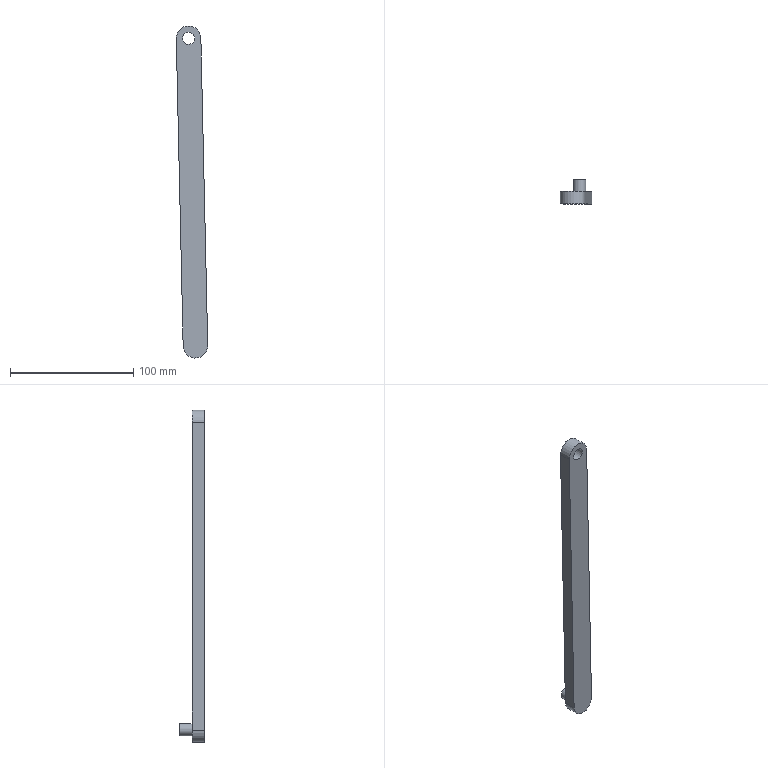Component | NX | 03 | 1 solid | 9 faces | box 25.59 x 20 x 269.94 mm | volume 53142 mm3 | plane 5 | cylinder 4 | commonest cylinder face diameters 20 x2 10 x2
STEP:
#1=CARTESIAN_POINT('',(0.,0.,0.));
#2=DIRECTION('',(0.,0.,1.));
#3=DIRECTION('',(1.,0.,0.));
#4=AXIS2_PLACEMENT_3D('',#1,#2,#3);
#5=CARTESIAN_POINT('',(208.953,15.,299.814));
#6=VERTEX_POINT('',#5);
#7=CARTESIAN_POINT('',(188.958,15.,299.367));
#8=VERTEX_POINT('',#7);
#9=CARTESIAN_POINT('',(198.956,15.,299.59));
#10=DIRECTION('',(0.,-1.,0.));
#11=DIRECTION('',(0.02235,0.,-0.9998));
#12=AXIS2_PLACEMENT_3D('',#9,#10,#11);
#13=CIRCLE('',#12,10.);
#14=CARTESIAN_POINT('',(198.956,5.,299.59));
#15=DIRECTION('',(0.,1.,0.));
#16=DIRECTION('',(0.9998,0.,0.02235));
#17=AXIS2_PLACEMENT_3D('',#14,#15,#16);
#18=CYLINDRICAL_SURFACE('',#17,10.);
#19=CARTESIAN_POINT('',(7.854,10.));
#20=DIRECTION('',(-1.,0.));
#21=VECTOR('',#20,1.);
#22=LINE('',#19,#21);
#23=(GEOMETRIC_REPRESENTATION_CONTEXT(2)PARAMETRIC_REPRESENTATION_CONTEXT()REPRESENTATION_CONTEXT('',''));
#24=DEFINITIONAL_REPRESENTATION('',(#22),#23);
#25=PCURVE('',#18,#24);
#26=CARTESIAN_POINT('',(198.956,15.,299.59));
#27=DIRECTION('',(0.,-1.,0.));
#28=DIRECTION('',(-0.9998,0.,-0.02235));
#29=AXIS2_PLACEMENT_3D('',#26,#27,#28);
#30=PLANE('',#29);
#31=CARTESIAN_POINT('',(0.,0.));
#32=DIRECTION('',(-0.,1.));
#33=AXIS2_PLACEMENT_2D('',#31,#32);
#34=CIRCLE('',#33,10.);
#35=(GEOMETRIC_REPRESENTATION_CONTEXT(2)PARAMETRIC_REPRESENTATION_CONTEXT()REPRESENTATION_CONTEXT('',''));
#36=DEFINITIONAL_REPRESENTATION('',(#34),#35);
#37=PCURVE('',#30,#36);
#38=SURFACE_CURVE('',#13,(#25,#37),.PCURVE_S1.);
#39=EDGE_CURVE('',#6,#8,#38,.T.);
#40=ORIENTED_EDGE('',*,*,#39,.T.);
#41=CARTESIAN_POINT('',(188.958,5.,299.367));
#42=VERTEX_POINT('',#41);
#43=CARTESIAN_POINT('',(188.958,5.,299.367));
#44=DIRECTION('',(0.,1.,0.));
#45=VECTOR('',#44,1.);
#46=LINE('',#43,#45);
#47=CARTESIAN_POINT('',(3.142,0.));
#48=DIRECTION('',(0.,1.));
#49=VECTOR('',#48,1.);
#50=LINE('',#47,#49);
#51=(GEOMETRIC_REPRESENTATION_CONTEXT(2)PARAMETRIC_REPRESENTATION_CONTEXT()REPRESENTATION_CONTEXT('',''));
#52=DEFINITIONAL_REPRESENTATION('',(#50),#51);
#53=PCURVE('',#18,#52);
#54=CARTESIAN_POINT('',(188.958,5.,299.367));
#55=DIRECTION('',(0.9998,0.,0.02235));
#56=DIRECTION('',(0.02235,0.,-0.9998));
#57=AXIS2_PLACEMENT_3D('',#54,#55,#56);
#58=PLANE('',#57);
#59=CARTESIAN_POINT('',(0.,0.));
#60=DIRECTION('',(0.,1.));
#61=VECTOR('',#60,1.);
#62=LINE('',#59,#61);
#63=(GEOMETRIC_REPRESENTATION_CONTEXT(2)PARAMETRIC_REPRESENTATION_CONTEXT()REPRESENTATION_CONTEXT('',''));
#64=DEFINITIONAL_REPRESENTATION('',(#62),#63);
#65=PCURVE('',#58,#64);
#66=SURFACE_CURVE('',#46,(#53,#65),.PCURVE_S1.);
#67=EDGE_CURVE('',#42,#8,#66,.T.);
#68=ORIENTED_EDGE('',*,*,#67,.F.);
#69=CARTESIAN_POINT('',(208.953,5.,299.814));
#70=VERTEX_POINT('',#69);
#71=CARTESIAN_POINT('',(198.956,5.,299.59));
#72=DIRECTION('',(0.,-1.,0.));
#73=DIRECTION('',(0.02235,0.,-0.9998));
#74=AXIS2_PLACEMENT_3D('',#71,#72,#73);
#75=CIRCLE('',#74,10.);
#76=CARTESIAN_POINT('',(7.854,0.));
#77=DIRECTION('',(-1.,0.));
#78=VECTOR('',#77,1.);
#79=LINE('',#76,#78);
#80=(GEOMETRIC_REPRESENTATION_CONTEXT(2)PARAMETRIC_REPRESENTATION_CONTEXT()REPRESENTATION_CONTEXT('',''));
#81=DEFINITIONAL_REPRESENTATION('',(#79),#80);
#82=PCURVE('',#18,#81);
#83=CARTESIAN_POINT('',(198.956,5.,299.59));
#84=DIRECTION('',(0.,-1.,0.));
#85=DIRECTION('',(-0.9998,0.,-0.02235));
#86=AXIS2_PLACEMENT_3D('',#83,#84,#85);
#87=PLANE('',#86);
#88=CARTESIAN_POINT('',(0.,0.));
#89=DIRECTION('',(-0.,1.));
#90=AXIS2_PLACEMENT_2D('',#88,#89);
#91=CIRCLE('',#90,10.);
#92=(GEOMETRIC_REPRESENTATION_CONTEXT(2)PARAMETRIC_REPRESENTATION_CONTEXT()REPRESENTATION_CONTEXT('',''));
#93=DEFINITIONAL_REPRESENTATION('',(#91),#92);
#94=PCURVE('',#87,#93);
#95=SURFACE_CURVE('',#75,(#82,#94),.PCURVE_S1.);
#96=EDGE_CURVE('',#70,#42,#95,.T.);
#97=ORIENTED_EDGE('',*,*,#96,.F.);
#98=CARTESIAN_POINT('',(208.953,5.,299.814));
#99=DIRECTION('',(0.,1.,0.));
#100=VECTOR('',#99,1.);
#101=LINE('',#98,#100);
#102=CARTESIAN_POINT('',(6.283,0.));
#103=DIRECTION('',(0.,1.));
#104=VECTOR('',#103,1.);
#105=LINE('',#102,#104);
#106=(GEOMETRIC_REPRESENTATION_CONTEXT(2)PARAMETRIC_REPRESENTATION_CONTEXT()REPRESENTATION_CONTEXT('',''));
#107=DEFINITIONAL_REPRESENTATION('',(#105),#106);
#108=PCURVE('',#18,#107);
#109=CARTESIAN_POINT('',(214.54,5.,49.876));
#110=DIRECTION('',(-0.9998,0.,-0.02235));
#111=DIRECTION('',(-0.02235,0.,0.9998));
#112=AXIS2_PLACEMENT_3D('',#109,#110,#111);
#113=PLANE('',#112);
#114=CARTESIAN_POINT('',(250.,0.));
#115=DIRECTION('',(0.,1.));
#116=VECTOR('',#115,1.);
#117=LINE('',#114,#116);
#118=(GEOMETRIC_REPRESENTATION_CONTEXT(2)PARAMETRIC_REPRESENTATION_CONTEXT()REPRESENTATION_CONTEXT('',''));
#119=DEFINITIONAL_REPRESENTATION('',(#117),#118);
#120=PCURVE('',#113,#119);
#121=SURFACE_CURVE('',#101,(#108,#120),.PCURVE_S1.);
#122=EDGE_CURVE('',#70,#6,#121,.T.);
#123=ORIENTED_EDGE('',*,*,#122,.T.);
#124=EDGE_LOOP('',(#40,#68,#97,#123));
#125=FACE_BOUND('',#124,.T.);
#126=ADVANCED_FACE('',(#125),#18,.T.);
#127=CARTESIAN_POINT('',(194.545,15.,49.429));
#128=VERTEX_POINT('',#127);
#129=CARTESIAN_POINT('',(188.958,15.,299.367));
#130=DIRECTION('',(0.02235,0.,-0.9998));
#131=VECTOR('',#130,1.);
#132=LINE('',#129,#131);
#133=CARTESIAN_POINT('',(0.,10.));
#134=DIRECTION('',(1.,0.));
#135=VECTOR('',#134,1.);
#136=LINE('',#133,#135);
#137=(GEOMETRIC_REPRESENTATION_CONTEXT(2)PARAMETRIC_REPRESENTATION_CONTEXT()REPRESENTATION_CONTEXT('',''));
#138=DEFINITIONAL_REPRESENTATION('',(#136),#137);
#139=PCURVE('',#58,#138);
#140=CARTESIAN_POINT('',(10.,-0.));
#141=DIRECTION('',(0.,1.));
#142=VECTOR('',#141,1.);
#143=LINE('',#140,#142);
#144=(GEOMETRIC_REPRESENTATION_CONTEXT(2)PARAMETRIC_REPRESENTATION_CONTEXT()REPRESENTATION_CONTEXT('',''));
#145=DEFINITIONAL_REPRESENTATION('',(#143),#144);
#146=PCURVE('',#30,#145);
#147=SURFACE_CURVE('',#132,(#139,#146),.PCURVE_S1.);
#148=EDGE_CURVE('',#8,#128,#147,.T.);
#149=ORIENTED_EDGE('',*,*,#148,.T.);
#150=CARTESIAN_POINT('',(194.545,5.,49.429));
#151=VERTEX_POINT('',#150);
#152=CARTESIAN_POINT('',(194.545,5.,49.429));
#153=DIRECTION('',(0.,1.,0.));
#154=VECTOR('',#153,1.);
#155=LINE('',#152,#154);
#156=CARTESIAN_POINT('',(250.,0.));
#157=DIRECTION('',(0.,1.));
#158=VECTOR('',#157,1.);
#159=LINE('',#156,#158);
#160=(GEOMETRIC_REPRESENTATION_CONTEXT(2)PARAMETRIC_REPRESENTATION_CONTEXT()REPRESENTATION_CONTEXT('',''));
#161=DEFINITIONAL_REPRESENTATION('',(#159),#160);
#162=PCURVE('',#58,#161);
#163=CARTESIAN_POINT('',(204.543,5.,49.653));
#164=DIRECTION('',(0.,1.,0.));
#165=DIRECTION('',(0.9998,0.,0.02235));
#166=AXIS2_PLACEMENT_3D('',#163,#164,#165);
#167=CYLINDRICAL_SURFACE('',#166,10.);
#168=CARTESIAN_POINT('',(3.142,0.));
#169=DIRECTION('',(0.,1.));
#170=VECTOR('',#169,1.);
#171=LINE('',#168,#170);
#172=(GEOMETRIC_REPRESENTATION_CONTEXT(2)PARAMETRIC_REPRESENTATION_CONTEXT()REPRESENTATION_CONTEXT('',''));
#173=DEFINITIONAL_REPRESENTATION('',(#171),#172);
#174=PCURVE('',#167,#173);
#175=SURFACE_CURVE('',#155,(#162,#174),.PCURVE_S1.);
#176=EDGE_CURVE('',#151,#128,#175,.T.);
#177=ORIENTED_EDGE('',*,*,#176,.F.);
#178=CARTESIAN_POINT('',(188.958,5.,299.367));
#179=DIRECTION('',(0.02235,0.,-0.9998));
#180=VECTOR('',#179,1.);
#181=LINE('',#178,#180);
#182=CARTESIAN_POINT('',(0.,0.));
#183=DIRECTION('',(1.,0.));
#184=VECTOR('',#183,1.);
#185=LINE('',#182,#184);
#186=(GEOMETRIC_REPRESENTATION_CONTEXT(2)PARAMETRIC_REPRESENTATION_CONTEXT()REPRESENTATION_CONTEXT('',''));
#187=DEFINITIONAL_REPRESENTATION('',(#185),#186);
#188=PCURVE('',#58,#187);
#189=CARTESIAN_POINT('',(10.,-0.));
#190=DIRECTION('',(0.,1.));
#191=VECTOR('',#190,1.);
#192=LINE('',#189,#191);
#193=(GEOMETRIC_REPRESENTATION_CONTEXT(2)PARAMETRIC_REPRESENTATION_CONTEXT()REPRESENTATION_CONTEXT('',''));
#194=DEFINITIONAL_REPRESENTATION('',(#192),#193);
#195=PCURVE('',#87,#194);
#196=SURFACE_CURVE('',#181,(#188,#195),.PCURVE_S1.);
#197=EDGE_CURVE('',#42,#151,#196,.T.);
#198=ORIENTED_EDGE('',*,*,#197,.F.);
#199=ORIENTED_EDGE('',*,*,#67,.T.);
#200=EDGE_LOOP('',(#149,#177,#198,#199));
#201=FACE_BOUND('',#200,.T.);
#202=ADVANCED_FACE('',(#201),#58,.F.);
#203=CARTESIAN_POINT('',(214.54,15.,49.876));
#204=VERTEX_POINT('',#203);
#205=CARTESIAN_POINT('',(204.543,15.,49.653));
#206=DIRECTION('',(0.,-1.,0.));
#207=DIRECTION('',(0.02235,0.,-0.9998));
#208=AXIS2_PLACEMENT_3D('',#205,#206,#207);
#209=CIRCLE('',#208,10.);
#210=CARTESIAN_POINT('',(7.854,10.));
#211=DIRECTION('',(-1.,0.));
#212=VECTOR('',#211,1.);
#213=LINE('',#210,#212);
#214=(GEOMETRIC_REPRESENTATION_CONTEXT(2)PARAMETRIC_REPRESENTATION_CONTEXT()REPRESENTATION_CONTEXT('',''));
#215=DEFINITIONAL_REPRESENTATION('',(#213),#214);
#216=PCURVE('',#167,#215);
#217=CARTESIAN_POINT('',(0.,250.));
#218=DIRECTION('',(-0.,1.));
#219=AXIS2_PLACEMENT_2D('',#217,#218);
#220=CIRCLE('',#219,10.);
#221=(GEOMETRIC_REPRESENTATION_CONTEXT(2)PARAMETRIC_REPRESENTATION_CONTEXT()REPRESENTATION_CONTEXT('',''));
#222=DEFINITIONAL_REPRESENTATION('',(#220),#221);
#223=PCURVE('',#30,#222);
#224=SURFACE_CURVE('',#209,(#216,#223),.PCURVE_S1.);
#225=EDGE_CURVE('',#128,#204,#224,.T.);
#226=ORIENTED_EDGE('',*,*,#225,.T.);
#227=CARTESIAN_POINT('',(214.54,5.,49.876));
#228=VERTEX_POINT('',#227);
#229=CARTESIAN_POINT('',(214.54,5.,49.876));
#230=DIRECTION('',(0.,1.,0.));
#231=VECTOR('',#230,1.);
#232=LINE('',#229,#231);
#233=CARTESIAN_POINT('',(0.,0.));
#234=DIRECTION('',(0.,1.));
#235=VECTOR('',#234,1.);
#236=LINE('',#233,#235);
#237=(GEOMETRIC_REPRESENTATION_CONTEXT(2)PARAMETRIC_REPRESENTATION_CONTEXT()REPRESENTATION_CONTEXT('',''));
#238=DEFINITIONAL_REPRESENTATION('',(#236),#237);
#239=PCURVE('',#167,#238);
#240=CARTESIAN_POINT('',(0.,0.));
#241=DIRECTION('',(0.,1.));
#242=VECTOR('',#241,1.);
#243=LINE('',#240,#242);
#244=(GEOMETRIC_REPRESENTATION_CONTEXT(2)PARAMETRIC_REPRESENTATION_CONTEXT()REPRESENTATION_CONTEXT('',''));
#245=DEFINITIONAL_REPRESENTATION('',(#243),#244);
#246=PCURVE('',#113,#245);
#247=SURFACE_CURVE('',#232,(#239,#246),.PCURVE_S1.);
#248=EDGE_CURVE('',#228,#204,#247,.T.);
#249=ORIENTED_EDGE('',*,*,#248,.F.);
#250=CARTESIAN_POINT('',(204.543,5.,49.653));
#251=DIRECTION('',(0.,-1.,0.));
#252=DIRECTION('',(0.02235,0.,-0.9998));
#253=AXIS2_PLACEMENT_3D('',#250,#251,#252);
#254=CIRCLE('',#253,10.);
#255=CARTESIAN_POINT('',(7.854,0.));
#256=DIRECTION('',(-1.,0.));
#257=VECTOR('',#256,1.);
#258=LINE('',#255,#257);
#259=(GEOMETRIC_REPRESENTATION_CONTEXT(2)PARAMETRIC_REPRESENTATION_CONTEXT()REPRESENTATION_CONTEXT('',''));
#260=DEFINITIONAL_REPRESENTATION('',(#258),#259);
#261=PCURVE('',#167,#260);
#262=CARTESIAN_POINT('',(0.,250.));
#263=DIRECTION('',(-0.,1.));
#264=AXIS2_PLACEMENT_2D('',#262,#263);
#265=CIRCLE('',#264,10.);
#266=(GEOMETRIC_REPRESENTATION_CONTEXT(2)PARAMETRIC_REPRESENTATION_CONTEXT()REPRESENTATION_CONTEXT('',''));
#267=DEFINITIONAL_REPRESENTATION('',(#265),#266);
#268=PCURVE('',#87,#267);
#269=SURFACE_CURVE('',#254,(#261,#268),.PCURVE_S1.);
#270=EDGE_CURVE('',#151,#228,#269,.T.);
#271=ORIENTED_EDGE('',*,*,#270,.F.);
#272=ORIENTED_EDGE('',*,*,#176,.T.);
#273=EDGE_LOOP('',(#226,#249,#271,#272));
#274=FACE_BOUND('',#273,.T.);
#275=ADVANCED_FACE('',(#274),#167,.T.);
#276=CARTESIAN_POINT('',(214.54,15.,49.876));
#277=DIRECTION('',(-0.02235,0.,0.9998));
#278=VECTOR('',#277,1.);
#279=LINE('',#276,#278);
#280=CARTESIAN_POINT('',(0.,10.));
#281=DIRECTION('',(1.,0.));
#282=VECTOR('',#281,1.);
#283=LINE('',#280,#282);
#284=(GEOMETRIC_REPRESENTATION_CONTEXT(2)PARAMETRIC_REPRESENTATION_CONTEXT()REPRESENTATION_CONTEXT('',''));
#285=DEFINITIONAL_REPRESENTATION('',(#283),#284);
#286=PCURVE('',#113,#285);
#287=CARTESIAN_POINT('',(-10.,250.));
#288=DIRECTION('',(0.,-1.));
#289=VECTOR('',#288,1.);
#290=LINE('',#287,#289);
#291=(GEOMETRIC_REPRESENTATION_CONTEXT(2)PARAMETRIC_REPRESENTATION_CONTEXT()REPRESENTATION_CONTEXT('',''));
#292=DEFINITIONAL_REPRESENTATION('',(#290),#291);
#293=PCURVE('',#30,#292);
#294=SURFACE_CURVE('',#279,(#286,#293),.PCURVE_S1.);
#295=EDGE_CURVE('',#204,#6,#294,.T.);
#296=ORIENTED_EDGE('',*,*,#295,.T.);
#297=ORIENTED_EDGE('',*,*,#122,.F.);
#298=CARTESIAN_POINT('',(214.54,5.,49.876));
#299=DIRECTION('',(-0.02235,0.,0.9998));
#300=VECTOR('',#299,1.);
#301=LINE('',#298,#300);
#302=CARTESIAN_POINT('',(0.,0.));
#303=DIRECTION('',(1.,0.));
#304=VECTOR('',#303,1.);
#305=LINE('',#302,#304);
#306=(GEOMETRIC_REPRESENTATION_CONTEXT(2)PARAMETRIC_REPRESENTATION_CONTEXT()REPRESENTATION_CONTEXT('',''));
#307=DEFINITIONAL_REPRESENTATION('',(#305),#306);
#308=PCURVE('',#113,#307);
#309=CARTESIAN_POINT('',(-10.,250.));
#310=DIRECTION('',(0.,-1.));
#311=VECTOR('',#310,1.);
#312=LINE('',#309,#311);
#313=(GEOMETRIC_REPRESENTATION_CONTEXT(2)PARAMETRIC_REPRESENTATION_CONTEXT()REPRESENTATION_CONTEXT('',''));
#314=DEFINITIONAL_REPRESENTATION('',(#312),#313);
#315=PCURVE('',#87,#314);
#316=SURFACE_CURVE('',#301,(#308,#315),.PCURVE_S1.);
#317=EDGE_CURVE('',#228,#70,#316,.T.);
#318=ORIENTED_EDGE('',*,*,#317,.F.);
#319=ORIENTED_EDGE('',*,*,#248,.T.);
#320=EDGE_LOOP('',(#296,#297,#318,#319));
#321=FACE_BOUND('',#320,.T.);
#322=ADVANCED_FACE('',(#321),#113,.F.);
#323=CARTESIAN_POINT('',(193.957,5.,299.479));
#324=VERTEX_POINT('',#323);
#325=CARTESIAN_POINT('',(198.956,5.,299.59));
#326=DIRECTION('',(0.,-1.,0.));
#327=DIRECTION('',(-0.9998,0.,-0.02235));
#328=AXIS2_PLACEMENT_3D('',#325,#326,#327);
#329=CIRCLE('',#328,5.);
#330=CARTESIAN_POINT('',(0.,0.));
#331=DIRECTION('',(1.,0.));
#332=AXIS2_PLACEMENT_2D('',#330,#331);
#333=CIRCLE('',#332,5.);
#334=(GEOMETRIC_REPRESENTATION_CONTEXT(2)PARAMETRIC_REPRESENTATION_CONTEXT()REPRESENTATION_CONTEXT('',''));
#335=DEFINITIONAL_REPRESENTATION('',(#333),#334);
#336=PCURVE('',#87,#335);
#337=CARTESIAN_POINT('',(198.956,4.,299.59));
#338=DIRECTION('',(0.,1.,0.));
#339=DIRECTION('',(0.02235,0.,-0.9998));
#340=AXIS2_PLACEMENT_3D('',#337,#338,#339);
#341=CYLINDRICAL_SURFACE('',#340,5.);
#342=CARTESIAN_POINT('',(7.854,1.));
#343=DIRECTION('',(-1.,0.));
#344=VECTOR('',#343,1.);
#345=LINE('',#342,#344);
#346=(GEOMETRIC_REPRESENTATION_CONTEXT(2)PARAMETRIC_REPRESENTATION_CONTEXT()REPRESENTATION_CONTEXT('',''));
#347=DEFINITIONAL_REPRESENTATION('',(#345),#346);
#348=PCURVE('',#341,#347);
#349=SURFACE_CURVE('',#329,(#336,#348),.PCURVE_S1.);
#350=EDGE_CURVE('',#324,#324,#349,.T.);
#351=ORIENTED_EDGE('',*,*,#350,.F.);
#352=EDGE_LOOP('',(#351));
#353=FACE_BOUND('',#352,.T.);
#354=ORIENTED_EDGE('',*,*,#96,.T.);
#355=ORIENTED_EDGE('',*,*,#197,.T.);
#356=ORIENTED_EDGE('',*,*,#270,.T.);
#357=ORIENTED_EDGE('',*,*,#317,.T.);
#358=EDGE_LOOP('',(#354,#355,#356,#357));
#359=FACE_BOUND('',#358,.T.);
#360=ADVANCED_FACE('',(#353,#359),#87,.T.);
#361=CARTESIAN_POINT('',(204.431,15.,54.652));
#362=VERTEX_POINT('',#361);
#363=CARTESIAN_POINT('',(204.543,15.,49.653));
#364=DIRECTION('',(0.,-1.,0.));
#365=DIRECTION('',(-0.02235,0.,0.9998));
#366=AXIS2_PLACEMENT_3D('',#363,#364,#365);
#367=CIRCLE('',#366,5.);
#368=CARTESIAN_POINT('',(0.,250.));
#369=DIRECTION('',(0.,-1.));
#370=AXIS2_PLACEMENT_2D('',#368,#369);
#371=CIRCLE('',#370,5.);
#372=(GEOMETRIC_REPRESENTATION_CONTEXT(2)PARAMETRIC_REPRESENTATION_CONTEXT()REPRESENTATION_CONTEXT('',''));
#373=DEFINITIONAL_REPRESENTATION('',(#371),#372);
#374=PCURVE('',#30,#373);
#375=CARTESIAN_POINT('',(204.543,25.,49.653));
#376=DIRECTION('',(0.,-1.,0.));
#377=DIRECTION('',(-0.9998,0.,-0.02235));
#378=AXIS2_PLACEMENT_3D('',#375,#376,#377);
#379=CYLINDRICAL_SURFACE('',#378,5.);
#380=CARTESIAN_POINT('',(4.712,10.));
#381=DIRECTION('',(1.,0.));
#382=VECTOR('',#381,1.);
#383=LINE('',#380,#382);
#384=(GEOMETRIC_REPRESENTATION_CONTEXT(2)PARAMETRIC_REPRESENTATION_CONTEXT()REPRESENTATION_CONTEXT('',''));
#385=DEFINITIONAL_REPRESENTATION('',(#383),#384);
#386=PCURVE('',#379,#385);
#387=SURFACE_CURVE('',#367,(#374,#386),.PCURVE_S1.);
#388=EDGE_CURVE('',#362,#362,#387,.T.);
#389=ORIENTED_EDGE('',*,*,#388,.T.);
#390=EDGE_LOOP('',(#389));
#391=FACE_BOUND('',#390,.T.);
#392=CARTESIAN_POINT('',(193.957,15.,299.479));
#393=VERTEX_POINT('',#392);
#394=CARTESIAN_POINT('',(198.956,15.,299.59));
#395=DIRECTION('',(0.,-1.,0.));
#396=DIRECTION('',(-0.9998,0.,-0.02235));
#397=AXIS2_PLACEMENT_3D('',#394,#395,#396);
#398=CIRCLE('',#397,5.);
#399=CARTESIAN_POINT('',(0.,0.));
#400=DIRECTION('',(1.,0.));
#401=AXIS2_PLACEMENT_2D('',#399,#400);
#402=CIRCLE('',#401,5.);
#403=(GEOMETRIC_REPRESENTATION_CONTEXT(2)PARAMETRIC_REPRESENTATION_CONTEXT()REPRESENTATION_CONTEXT('',''));
#404=DEFINITIONAL_REPRESENTATION('',(#402),#403);
#405=PCURVE('',#30,#404);
#406=CARTESIAN_POINT('',(7.854,11.));
#407=DIRECTION('',(-1.,0.));
#408=VECTOR('',#407,1.);
#409=LINE('',#406,#408);
#410=(GEOMETRIC_REPRESENTATION_CONTEXT(2)PARAMETRIC_REPRESENTATION_CONTEXT()REPRESENTATION_CONTEXT('',''));
#411=DEFINITIONAL_REPRESENTATION('',(#409),#410);
#412=PCURVE('',#341,#411);
#413=SURFACE_CURVE('',#398,(#405,#412),.PCURVE_S1.);
#414=EDGE_CURVE('',#393,#393,#413,.T.);
#415=ORIENTED_EDGE('',*,*,#414,.T.);
#416=EDGE_LOOP('',(#415));
#417=FACE_BOUND('',#416,.T.);
#418=ORIENTED_EDGE('',*,*,#39,.F.);
#419=ORIENTED_EDGE('',*,*,#295,.F.);
#420=ORIENTED_EDGE('',*,*,#225,.F.);
#421=ORIENTED_EDGE('',*,*,#148,.F.);
#422=EDGE_LOOP('',(#418,#419,#420,#421));
#423=FACE_BOUND('',#422,.T.);
#424=ADVANCED_FACE('',(#391,#417,#423),#30,.F.);
#425=CARTESIAN_POINT('',(204.431,25.,54.652));
#426=VERTEX_POINT('',#425);
#427=CARTESIAN_POINT('',(204.543,25.,49.653));
#428=DIRECTION('',(0.,-1.,0.));
#429=DIRECTION('',(-0.02235,0.,0.9998));
#430=AXIS2_PLACEMENT_3D('',#427,#428,#429);
#431=CIRCLE('',#430,5.);
#432=CARTESIAN_POINT('',(4.712,0.));
#433=DIRECTION('',(1.,0.));
#434=VECTOR('',#433,1.);
#435=LINE('',#432,#434);
#436=(GEOMETRIC_REPRESENTATION_CONTEXT(2)PARAMETRIC_REPRESENTATION_CONTEXT()REPRESENTATION_CONTEXT('',''));
#437=DEFINITIONAL_REPRESENTATION('',(#435),#436);
#438=PCURVE('',#379,#437);
#439=CARTESIAN_POINT('',(204.543,25.,49.653));
#440=DIRECTION('',(0.,-1.,0.));
#441=DIRECTION('',(-0.9998,0.,-0.02235));
#442=AXIS2_PLACEMENT_3D('',#439,#440,#441);
#443=PLANE('',#442);
#444=CARTESIAN_POINT('',(0.,0.));
#445=DIRECTION('',(0.,-1.));
#446=AXIS2_PLACEMENT_2D('',#444,#445);
#447=CIRCLE('',#446,5.);
#448=(GEOMETRIC_REPRESENTATION_CONTEXT(2)PARAMETRIC_REPRESENTATION_CONTEXT()REPRESENTATION_CONTEXT('',''));
#449=DEFINITIONAL_REPRESENTATION('',(#447),#448);
#450=PCURVE('',#443,#449);
#451=SURFACE_CURVE('',#431,(#438,#450),.PCURVE_S1.);
#452=EDGE_CURVE('',#426,#426,#451,.T.);
#453=ORIENTED_EDGE('',*,*,#452,.T.);
#454=CARTESIAN_POINT('',(204.431,25.,54.652));
#455=CARTESIAN_POINT('',(204.431,15.,54.652));
#456=B_SPLINE_CURVE_WITH_KNOTS('',1,(#454,#455),.UNSPECIFIED.,.F.,.F.,(2,2),(0.,10.),.PIECEWISE_BEZIER_KNOTS.);
#457=CARTESIAN_POINT('',(10.996,0.));
#458=DIRECTION('',(0.,1.));
#459=VECTOR('',#458,1.);
#460=LINE('',#457,#459);
#461=(GEOMETRIC_REPRESENTATION_CONTEXT(2)PARAMETRIC_REPRESENTATION_CONTEXT()REPRESENTATION_CONTEXT('',''));
#462=DEFINITIONAL_REPRESENTATION('',(#460),#461);
#463=PCURVE('',#379,#462);
#464=CARTESIAN_POINT('',(4.712,0.));
#465=DIRECTION('',(0.,1.));
#466=VECTOR('',#465,1.);
#467=LINE('',#464,#466);
#468=(GEOMETRIC_REPRESENTATION_CONTEXT(2)PARAMETRIC_REPRESENTATION_CONTEXT()REPRESENTATION_CONTEXT('',''));
#469=DEFINITIONAL_REPRESENTATION('',(#467),#468);
#470=PCURVE('',#379,#469);
#471=SEAM_CURVE('',#456,(#463,#470),.PCURVE_S1.);
#472=EDGE_CURVE('',#426,#362,#471,.T.);
#473=ORIENTED_EDGE('',*,*,#472,.T.);
#474=ORIENTED_EDGE('',*,*,#388,.F.);
#475=ORIENTED_EDGE('',*,*,#472,.F.);
#476=EDGE_LOOP('',(#453,#473,#474,#475));
#477=FACE_BOUND('',#476,.T.);
#478=ADVANCED_FACE('',(#477),#379,.T.);
#479=ORIENTED_EDGE('',*,*,#452,.F.);
#480=EDGE_LOOP('',(#479));
#481=FACE_BOUND('',#480,.T.);
#482=ADVANCED_FACE('',(#481),#443,.F.);
#483=ORIENTED_EDGE('',*,*,#350,.F.);
#484=CARTESIAN_POINT('',(193.957,5.,299.479));
#485=CARTESIAN_POINT('',(193.957,15.,299.479));
#486=B_SPLINE_CURVE_WITH_KNOTS('',1,(#484,#485),.UNSPECIFIED.,.F.,.F.,(2,2),(1.,11.),.PIECEWISE_BEZIER_KNOTS.);
#487=CARTESIAN_POINT('',(7.854,0.));
#488=DIRECTION('',(0.,1.));
#489=VECTOR('',#488,1.);
#490=LINE('',#487,#489);
#491=(GEOMETRIC_REPRESENTATION_CONTEXT(2)PARAMETRIC_REPRESENTATION_CONTEXT()REPRESENTATION_CONTEXT('',''));
#492=DEFINITIONAL_REPRESENTATION('',(#490),#491);
#493=PCURVE('',#341,#492);
#494=CARTESIAN_POINT('',(1.571,0.));
#495=DIRECTION('',(0.,1.));
#496=VECTOR('',#495,1.);
#497=LINE('',#494,#496);
#498=(GEOMETRIC_REPRESENTATION_CONTEXT(2)PARAMETRIC_REPRESENTATION_CONTEXT()REPRESENTATION_CONTEXT('',''));
#499=DEFINITIONAL_REPRESENTATION('',(#497),#498);
#500=PCURVE('',#341,#499);
#501=SEAM_CURVE('',#486,(#493,#500),.PCURVE_S1.);
#502=EDGE_CURVE('',#324,#393,#501,.T.);
#503=ORIENTED_EDGE('',*,*,#502,.T.);
#504=ORIENTED_EDGE('',*,*,#414,.T.);
#505=ORIENTED_EDGE('',*,*,#502,.F.);
#506=EDGE_LOOP('',(#483,#503,#504,#505));
#507=FACE_BOUND('',#506,.F.);
#508=ADVANCED_FACE('',(#507),#341,.F.);
#509=CLOSED_SHELL('',(#126,#202,#275,#322,#360,#424,#478,#482,#508));
#510=MANIFOLD_SOLID_BREP('',#509);
#511=(LENGTH_UNIT()NAMED_UNIT(*)SI_UNIT(.MILLI.,.METRE.));
#512=UNCERTAINTY_MEASURE_WITH_UNIT(LENGTH_MEASURE(0.000002),#511,'','');
#513=(NAMED_UNIT(*)PLANE_ANGLE_UNIT()SI_UNIT($,.RADIAN.));
#514=(NAMED_UNIT(*)SI_UNIT($,.STERADIAN.)SOLID_ANGLE_UNIT());
#515=(GEOMETRIC_REPRESENTATION_CONTEXT(3)GLOBAL_UNCERTAINTY_ASSIGNED_CONTEXT((#512))GLOBAL_UNIT_ASSIGNED_CONTEXT((#511,#513,#514))REPRESENTATION_CONTEXT('',''));
#516=ADVANCED_BREP_SHAPE_REPRESENTATION('',(#4,#510),#515);